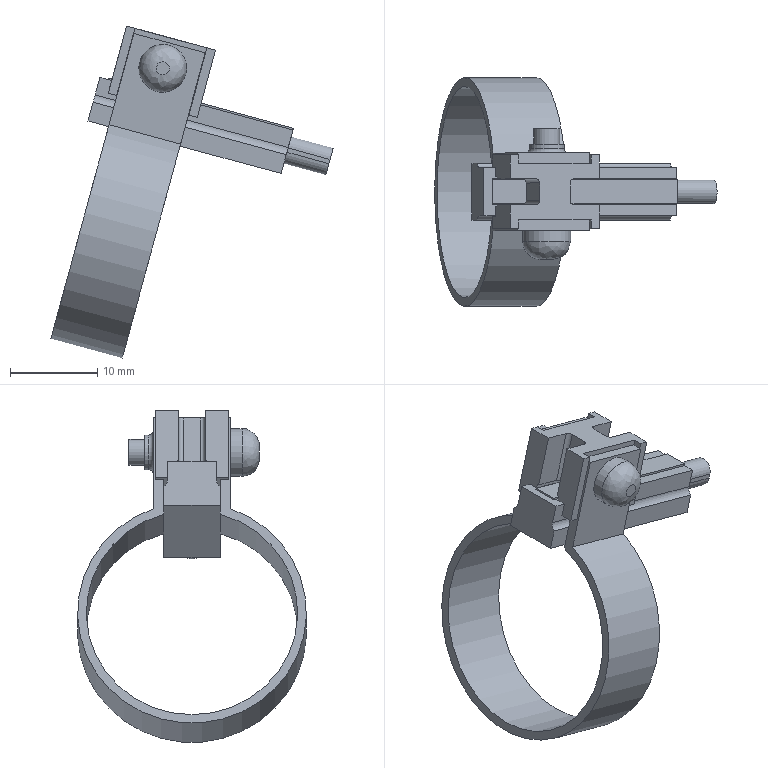Component | NX | DMSG | 1 solid | 81 faces | volume 2043 mm3 | plane 64 | cylinder 15 | torus 1 | spline 1 | commonest cylinder face diameters 1 x4 4 x3 2.7 x2 2 x2 5.5 x1 3 x1 26.3 x1 24.3 x1